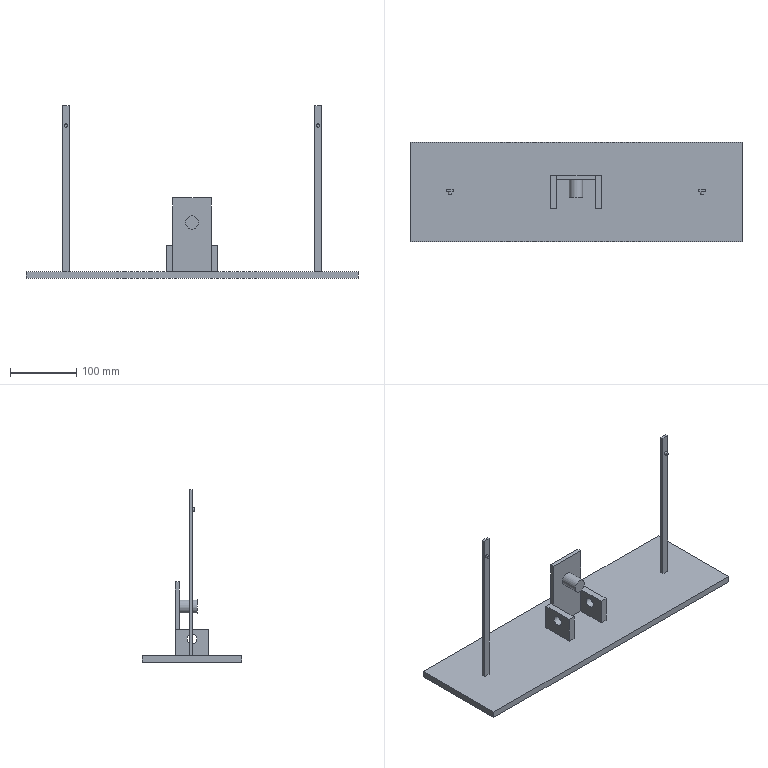Component | NX | BASE_PLATE | 1 solid | 37 faces | volume 853733 mm3 | plane 32 | cylinder 5 | commonest cylinder face diameters 15 x2 5 x2 20 x1